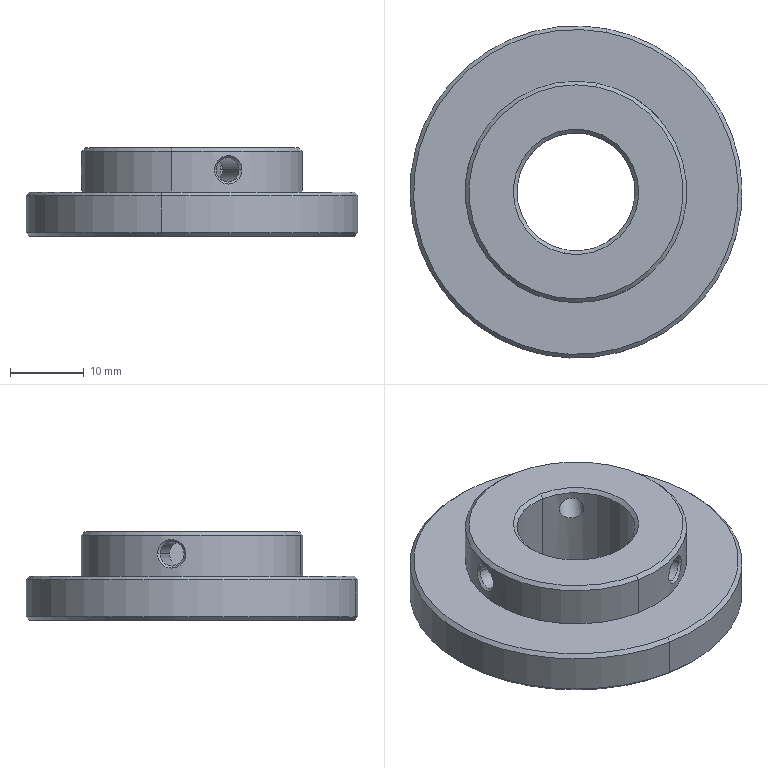Component | SolidWorks | YX-04-105GluePaperFeedingSensingBlock-1 | 1 solid | 31 faces | volume 11129 mm3 | cylinder 12 | cone 10 | spline 6 | plane 3 | commonest cylinder face diameters 3.3 x6 16 x2 30 x2 45 x2 | material 45#Steel